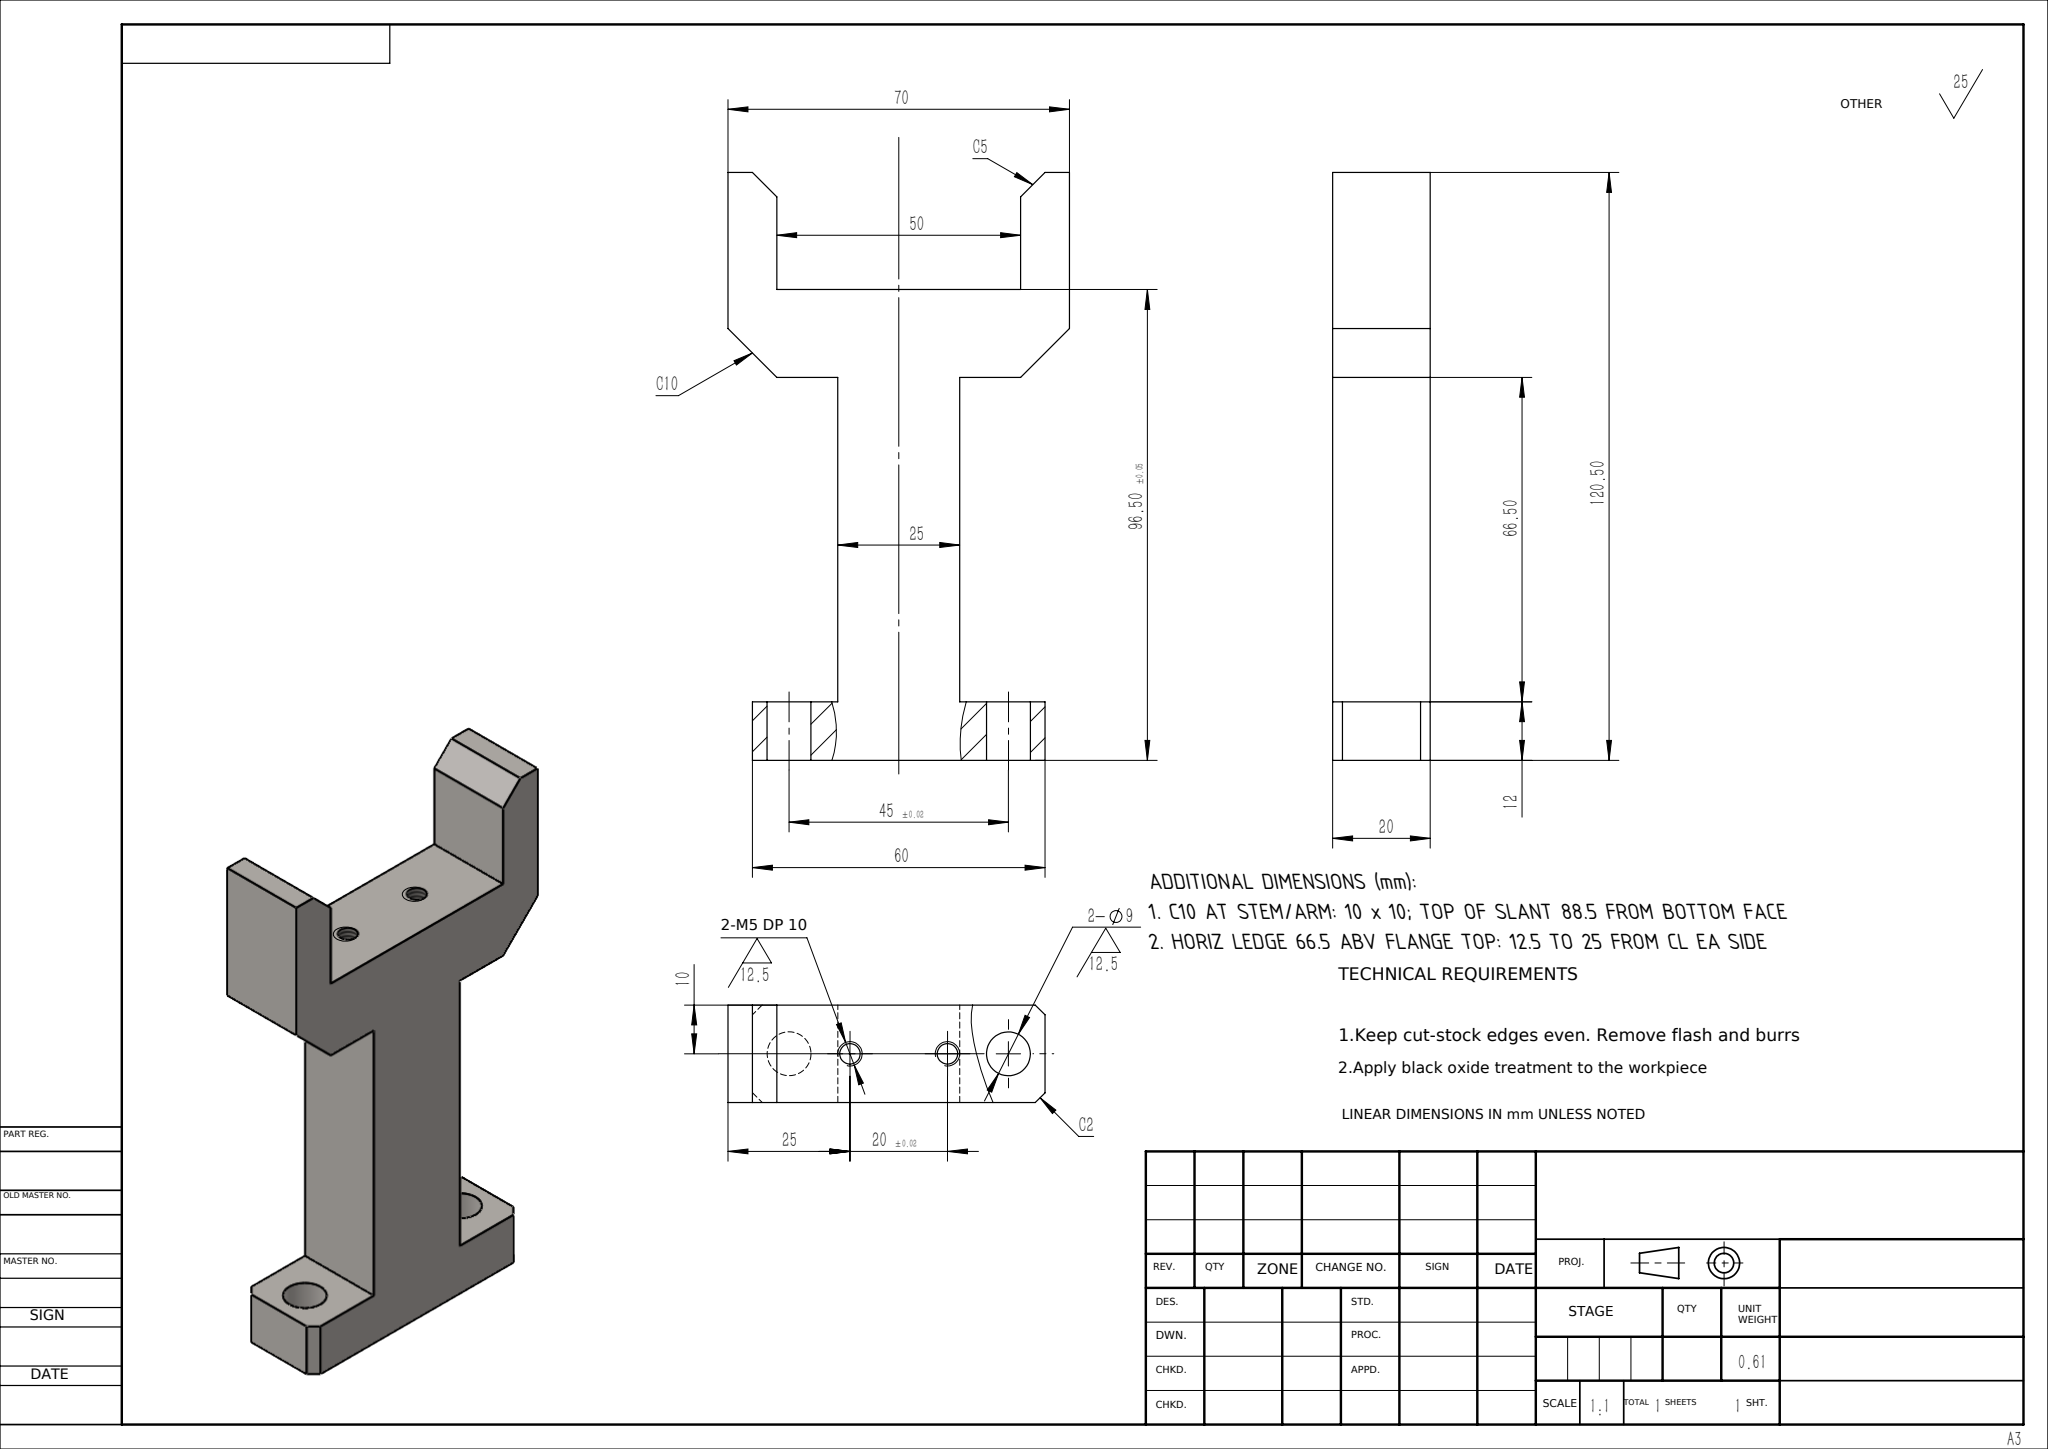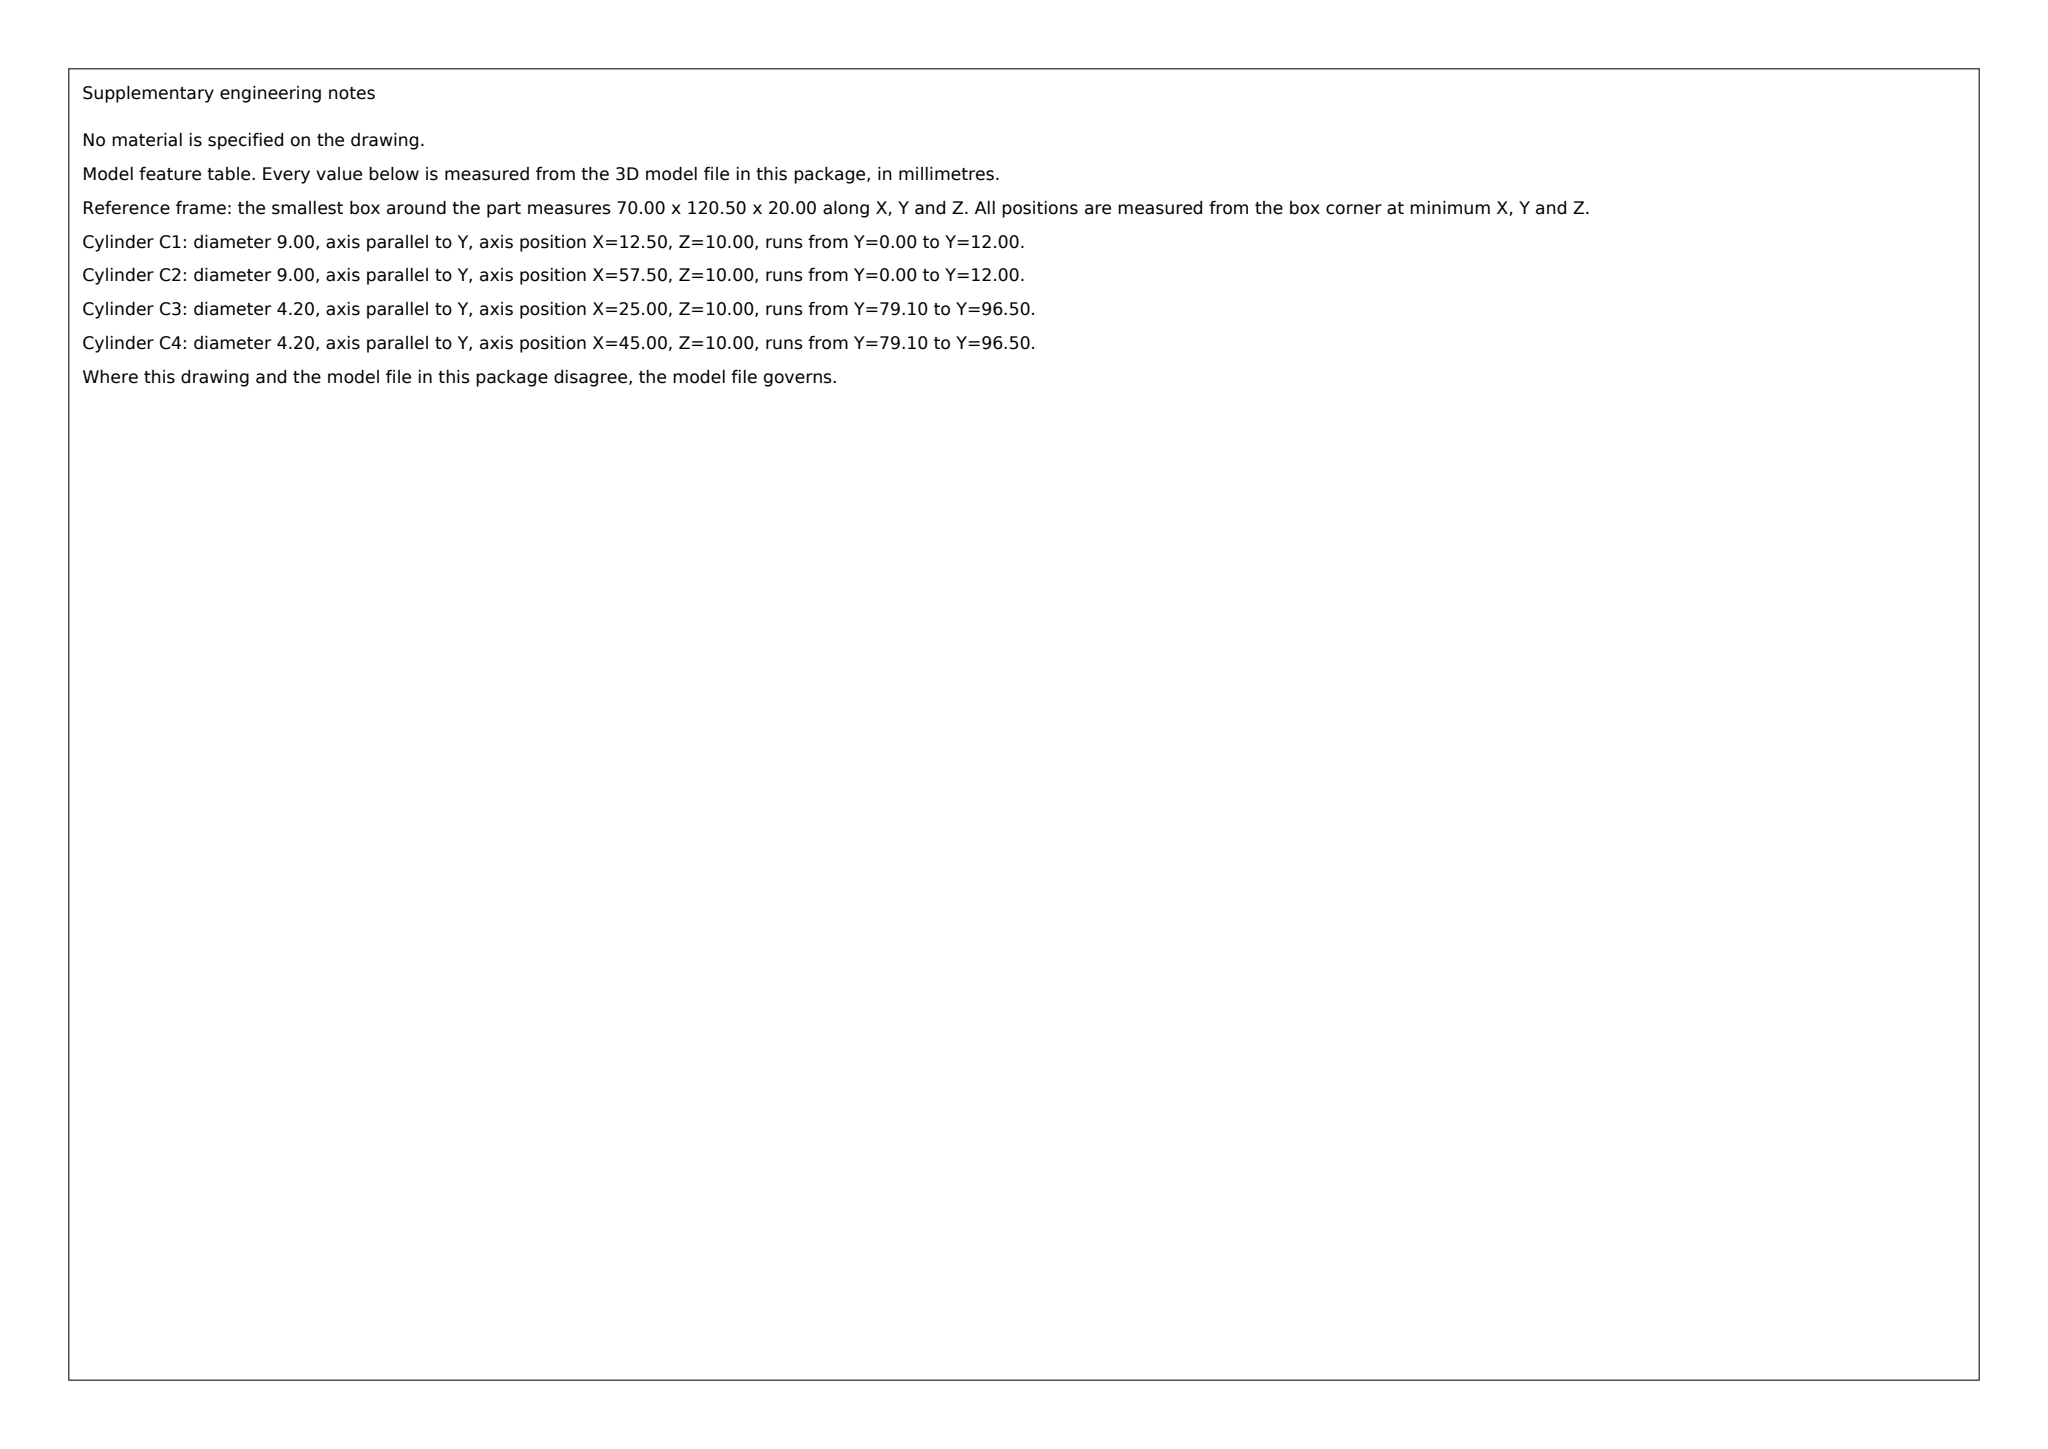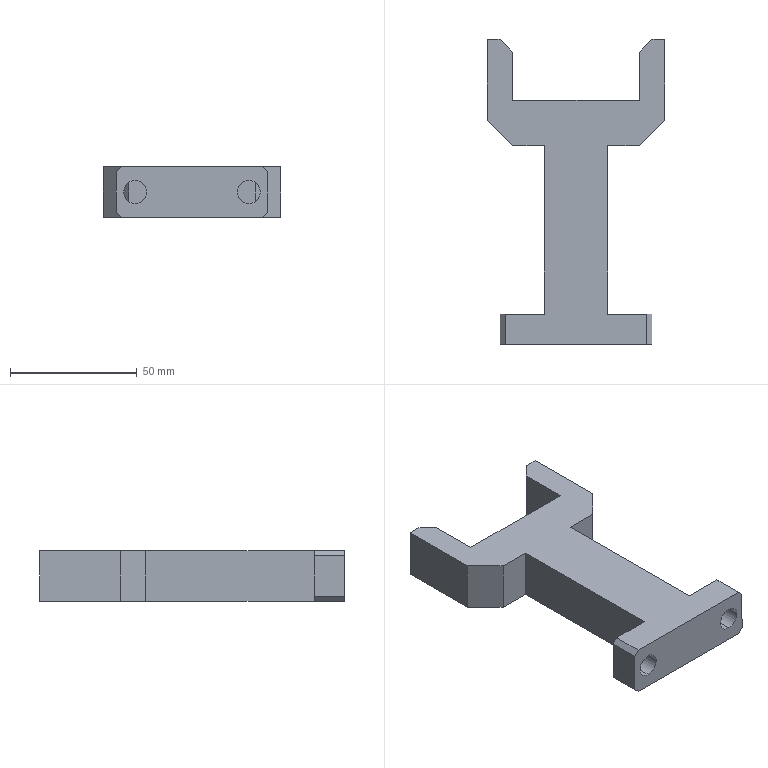Part | SolidWorks | mm | 1 solid | 38 faces | box 70 x 120.5 x 20 mm | volume 77833 mm3 | plane 26 | cylinder 8 | cone 4 | commonest cylinder face diameters 4.2 x4 9 x4
build123d program:
from build123d import *

# Parameters (mm, degrees)
BOSS_EXTRUDE1_DEPTH   = 10
CHAMFER1_SIZE         = 2
SKETCH3_R             = 4.5
CUT_EXTRUDE2_DEPTH    = 30
CHAMFER2_SIZE         = 10
CHAMFER3_SIZE         = 5
M5_TAPPED_HOLE1_D     = 4.2
M5_TAPPED_HOLE1_DEPTH = 17.4
M5_TAPPED_HOLE1_TIP   = 1.262


with BuildPart() as part:
    # Sketch1 → Boss-Extrude1 (new, symmetric)
    with BuildSketch(Plane.XY):
        Polygon((-30, 0), (30, 0), (30, 12), (12.5, 12), (12.5, 78.5), (35, 78.5), (35, 120.5), (25, 120.5), (25, 96.5), (-25, 96.5), (-25, 120.5), (-35, 120.5), (-35, 78.5), (-12.5, 78.5), (-12.5, 12), (-30, 12), align=None)
    extrude(amount=BOSS_EXTRUDE1_DEPTH, both=True)

    # Chamfer1
    chamfer1_edges = [part.edges().sort_by_distance(p)[0] for p in [
        (30, 6, 10),
        (30, 6, -10),
        (-30, 6, -10),
        (-30, 6, 10),
    ]]
    chamfer(chamfer1_edges, length=CHAMFER1_SIZE)

    # Sketch3 → Cut-Extrude2 (cut)
    with BuildSketch(Plane.XZ):
        with Locations(Location((22.5, 0, 0), (0, 0, 270))):
            Circle(SKETCH3_R)
        with Locations((-22.5, 0)):
            Circle(SKETCH3_R)
    extrude(amount=-CUT_EXTRUDE2_DEPTH, mode=Mode.SUBTRACT)

    # Chamfer2
    chamfer2_edges = [part.edges().sort_by_distance(p)[0] for p in [
        (-35, 78.5, 0),
        (35, 78.5, 0),
    ]]
    chamfer(chamfer2_edges, length=CHAMFER2_SIZE)

    # Chamfer3
    chamfer3_edges = [part.edges().sort_by_distance(p)[0] for p in [
        (-25, 120.5, 0),
        (25, 120.5, 0),
    ]]
    chamfer(chamfer3_edges, length=CHAMFER3_SIZE)

    # M5 Tapped Hole1
    with Locations(Plane(origin=(0, 96.5, 0), x_dir=(1, 0, 0), z_dir=(0, 1, 0))):
        with Locations((-10, 0), (10, 0)):
            Hole(M5_TAPPED_HOLE1_D / 2, depth=M5_TAPPED_HOLE1_DEPTH)
            with Locations((0, 0, -(M5_TAPPED_HOLE1_DEPTH + M5_TAPPED_HOLE1_TIP / 2))):  # 118° drill point
                Cone(0, M5_TAPPED_HOLE1_D / 2, M5_TAPPED_HOLE1_TIP, mode=Mode.SUBTRACT)


solid = part.part